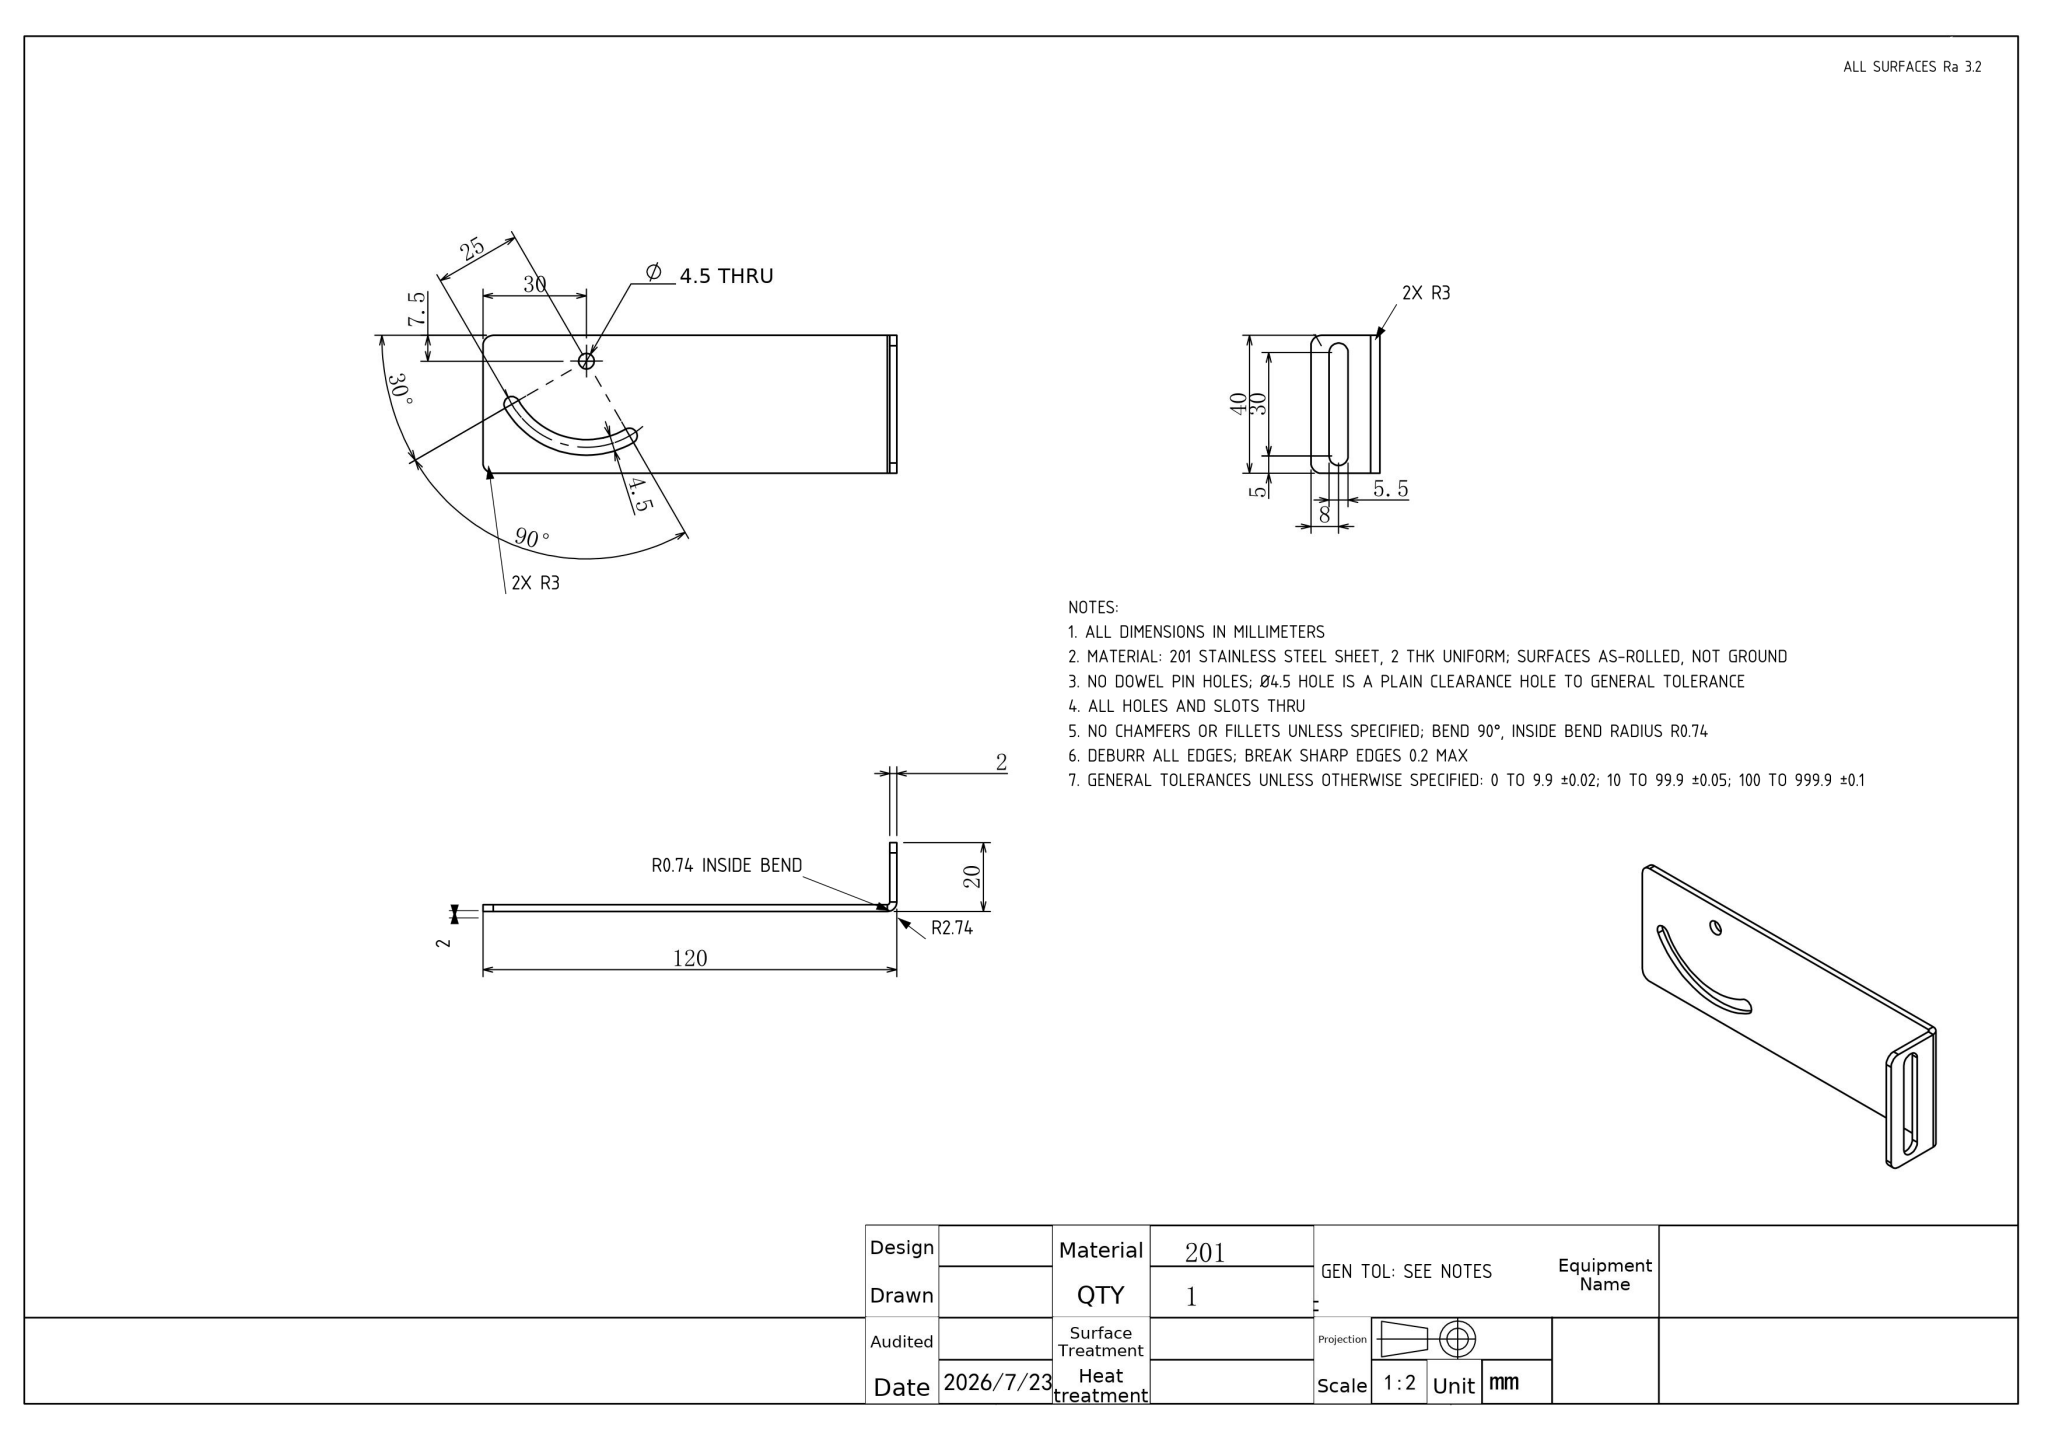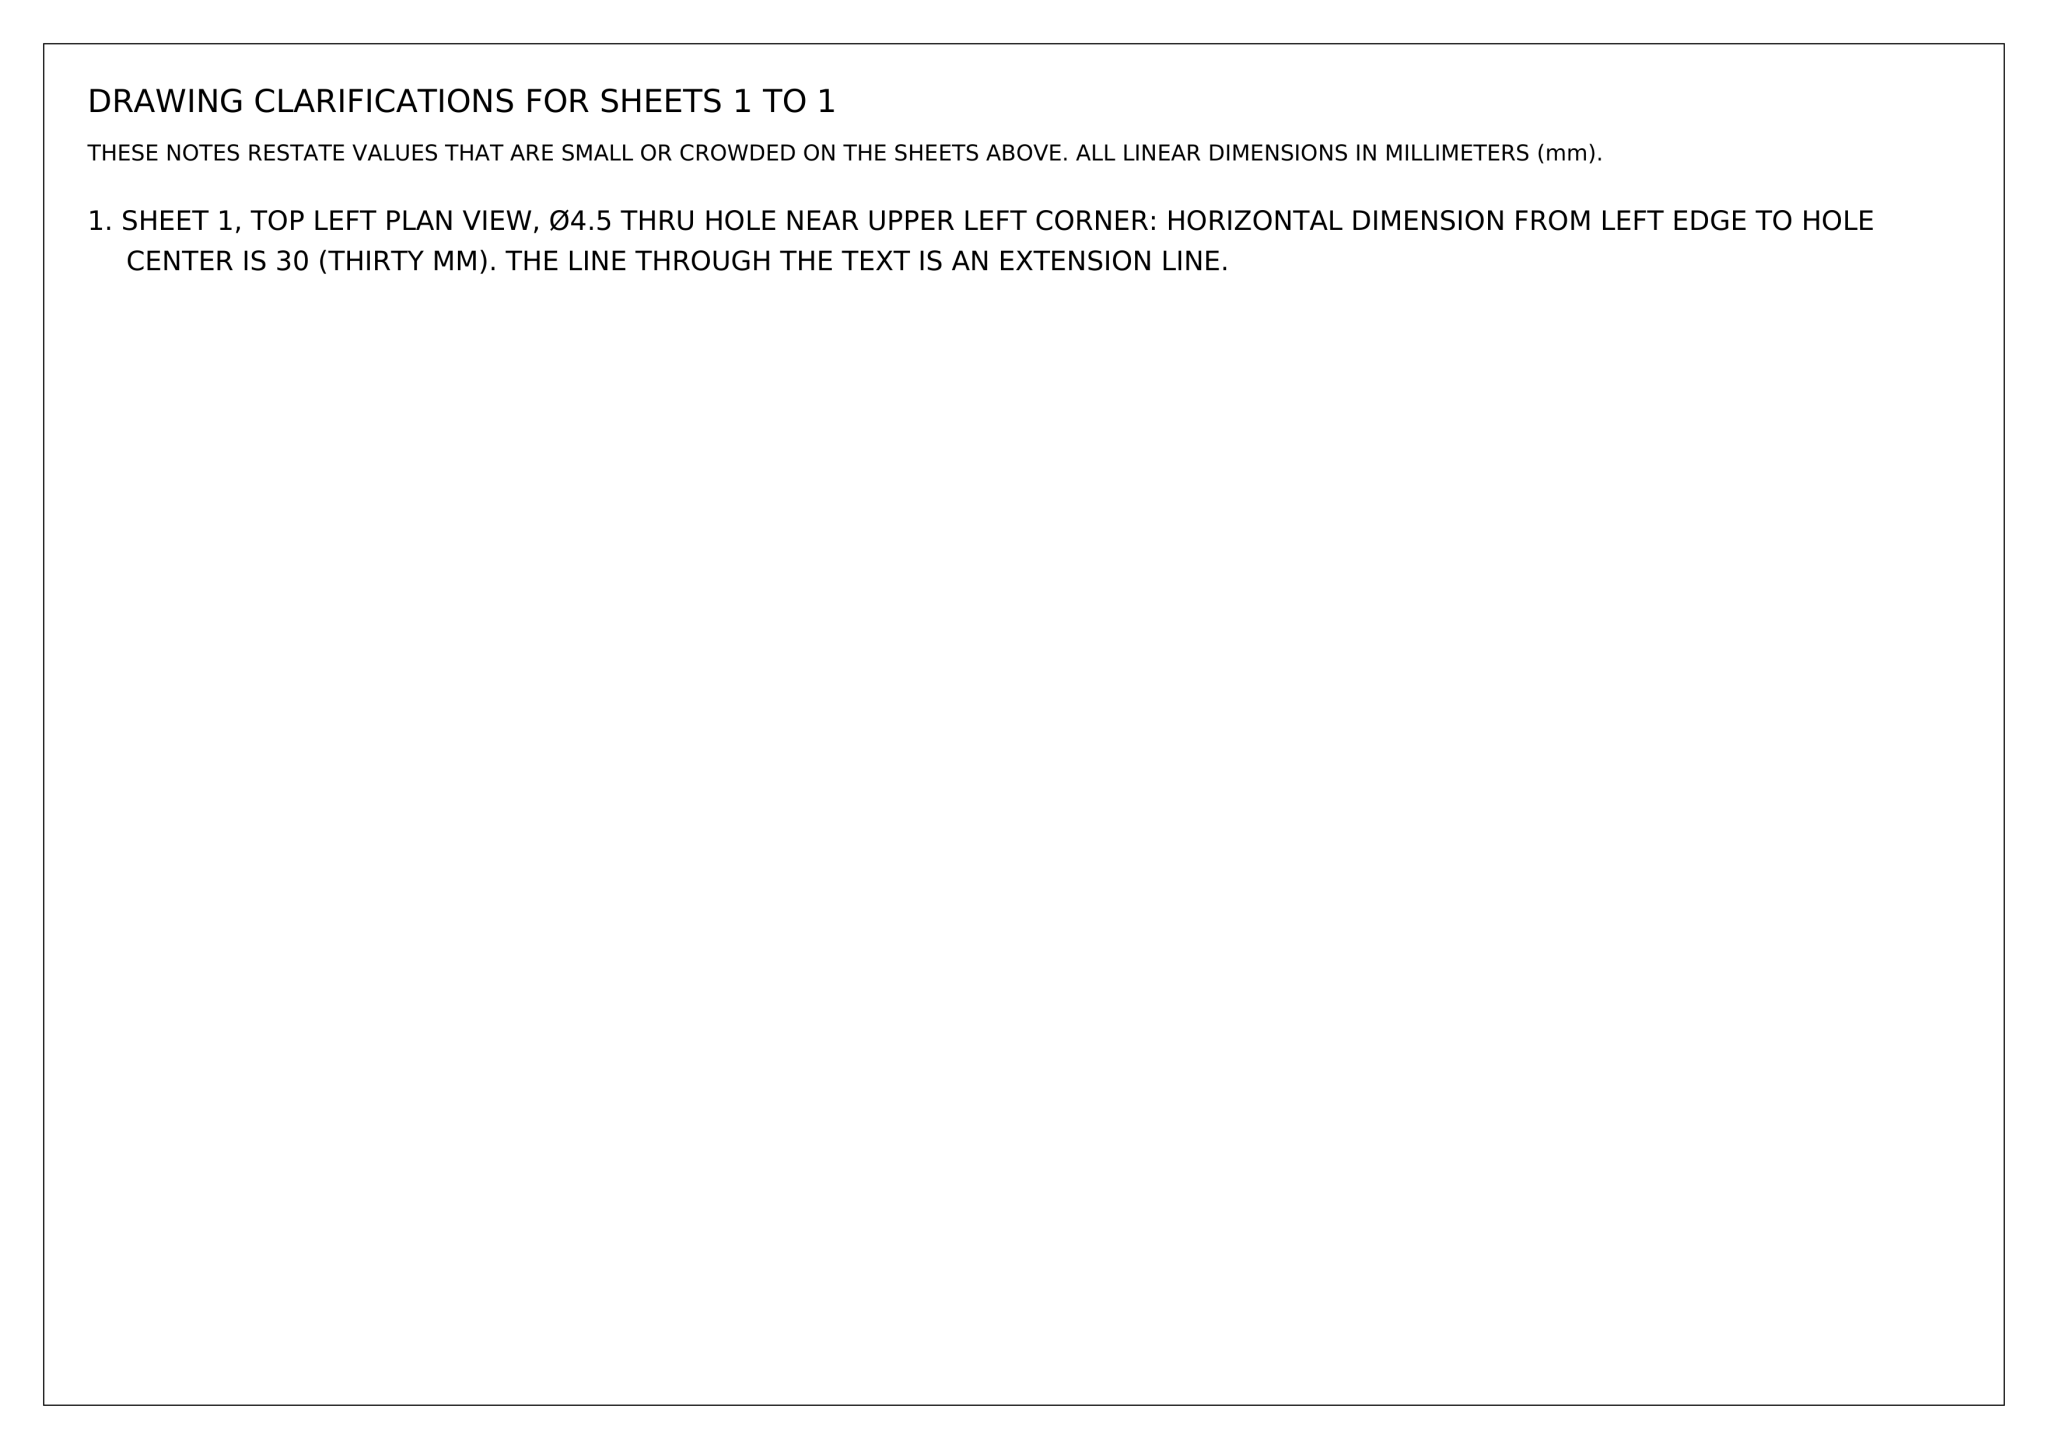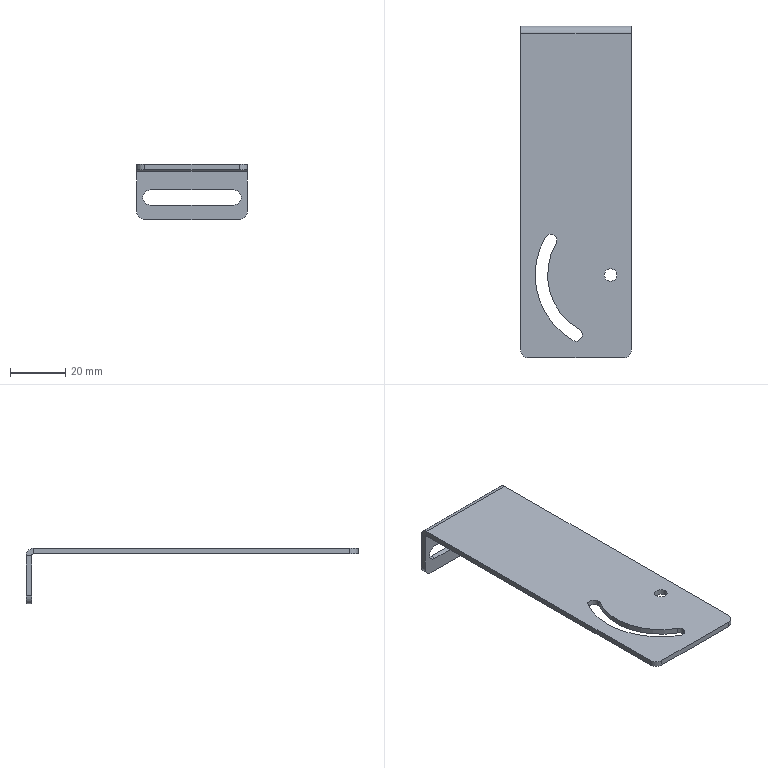Part | NX | mm | 1 solid | 30 faces | box 40 x 120 x 20 mm | volume 10170 mm3 | cylinder 16 | plane 14 | commonest cylinder face diameters 4.5 x6 6 x4 5.5 x2 5.473 x1 1.473 x1 45.5 x1 54.5 x1